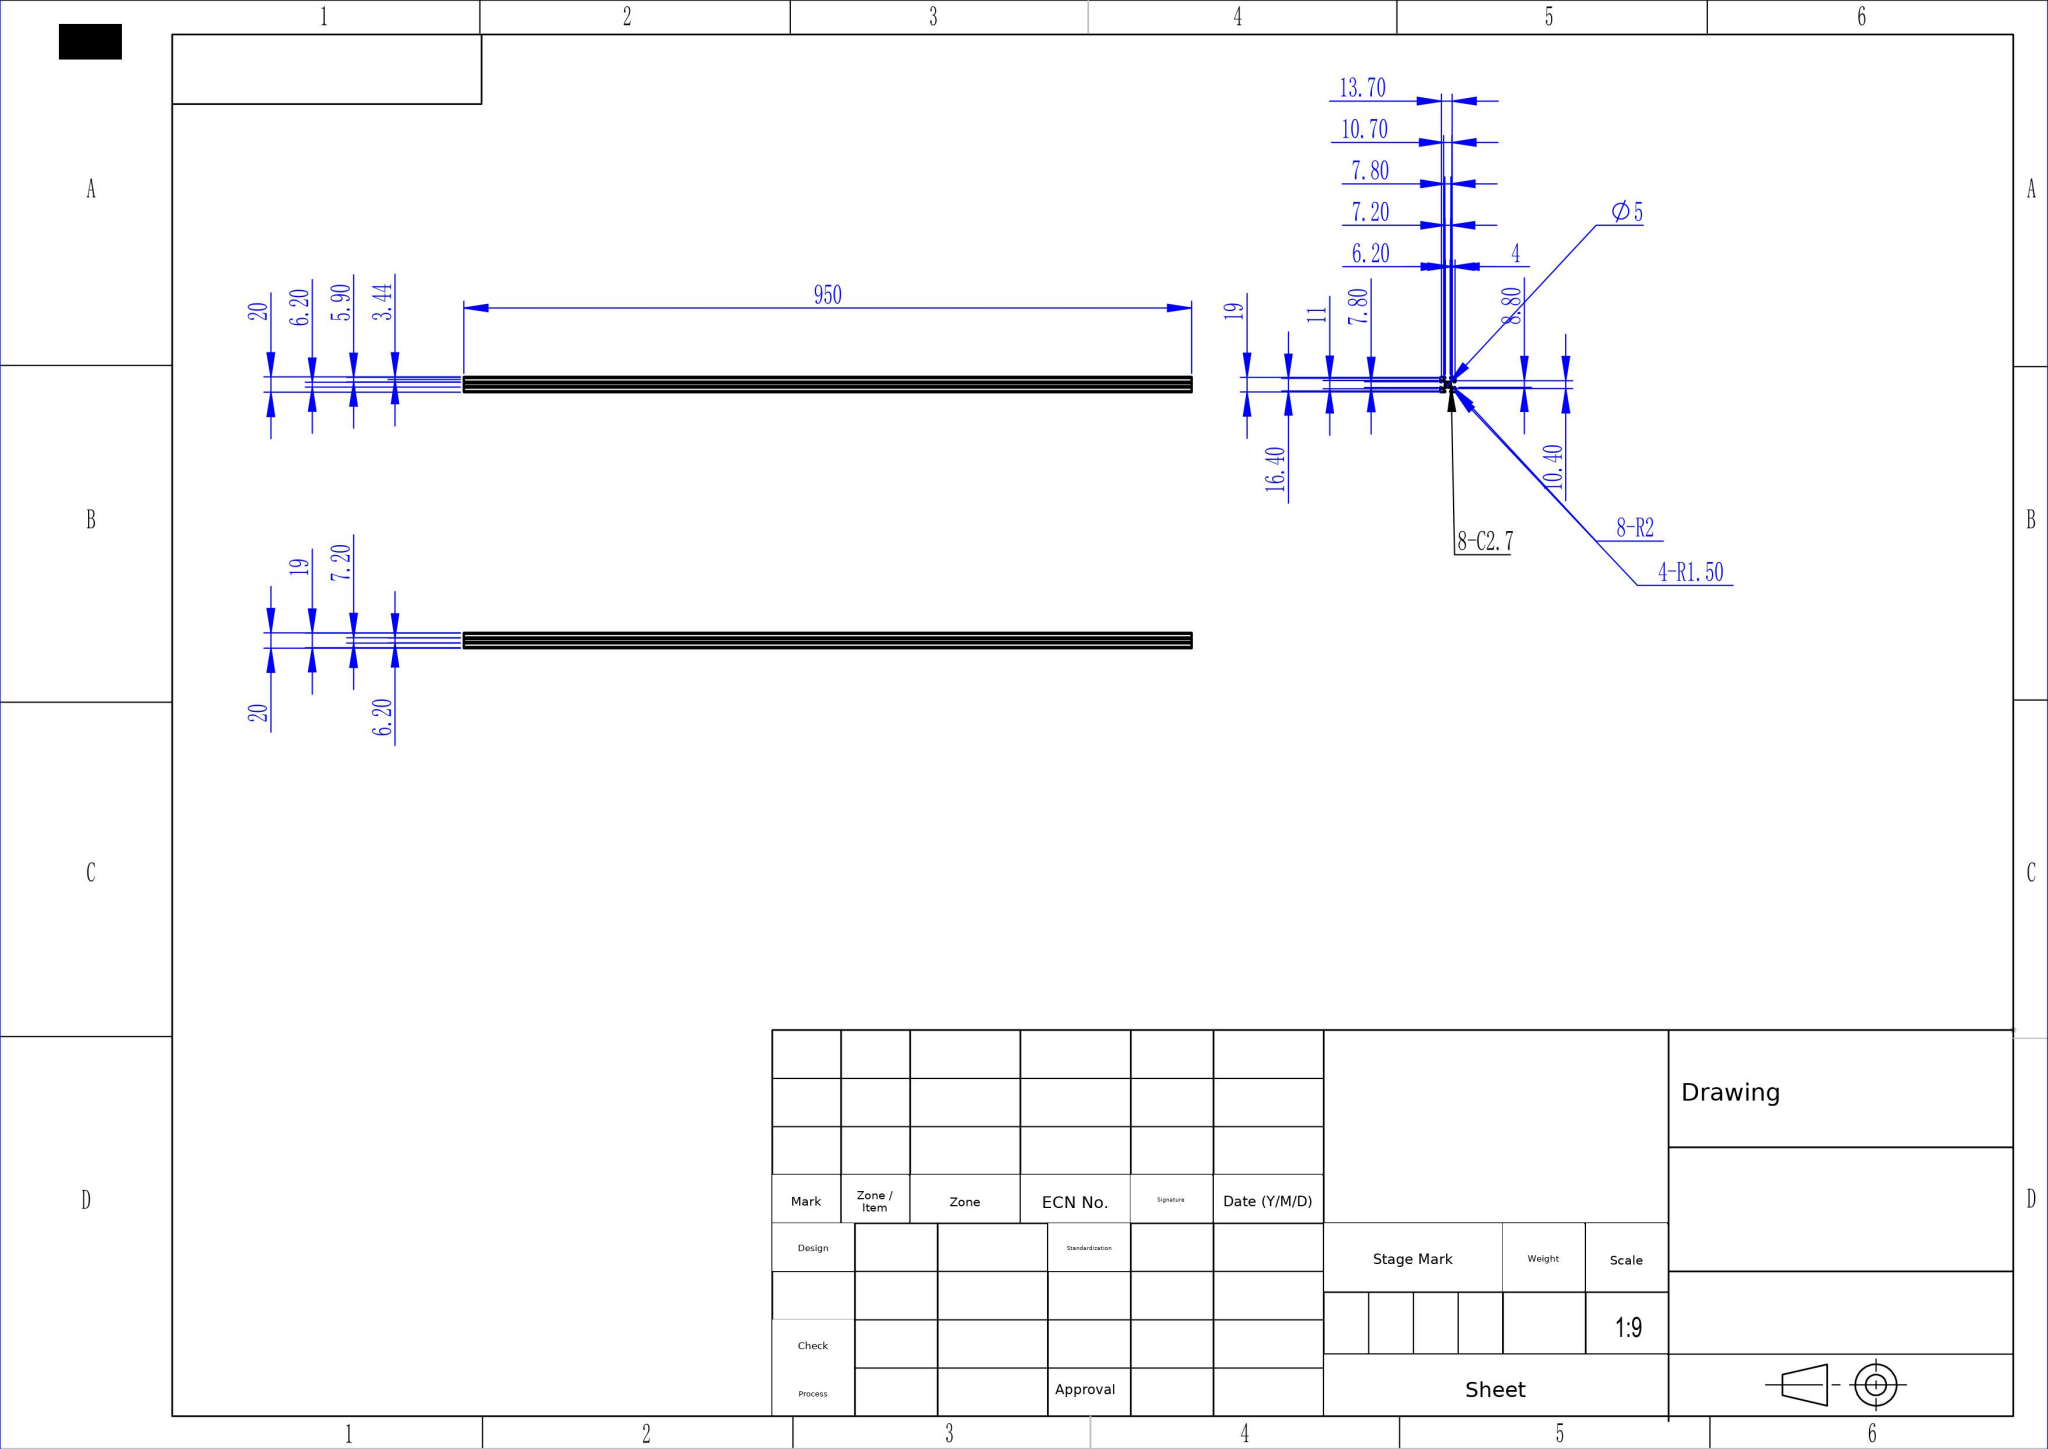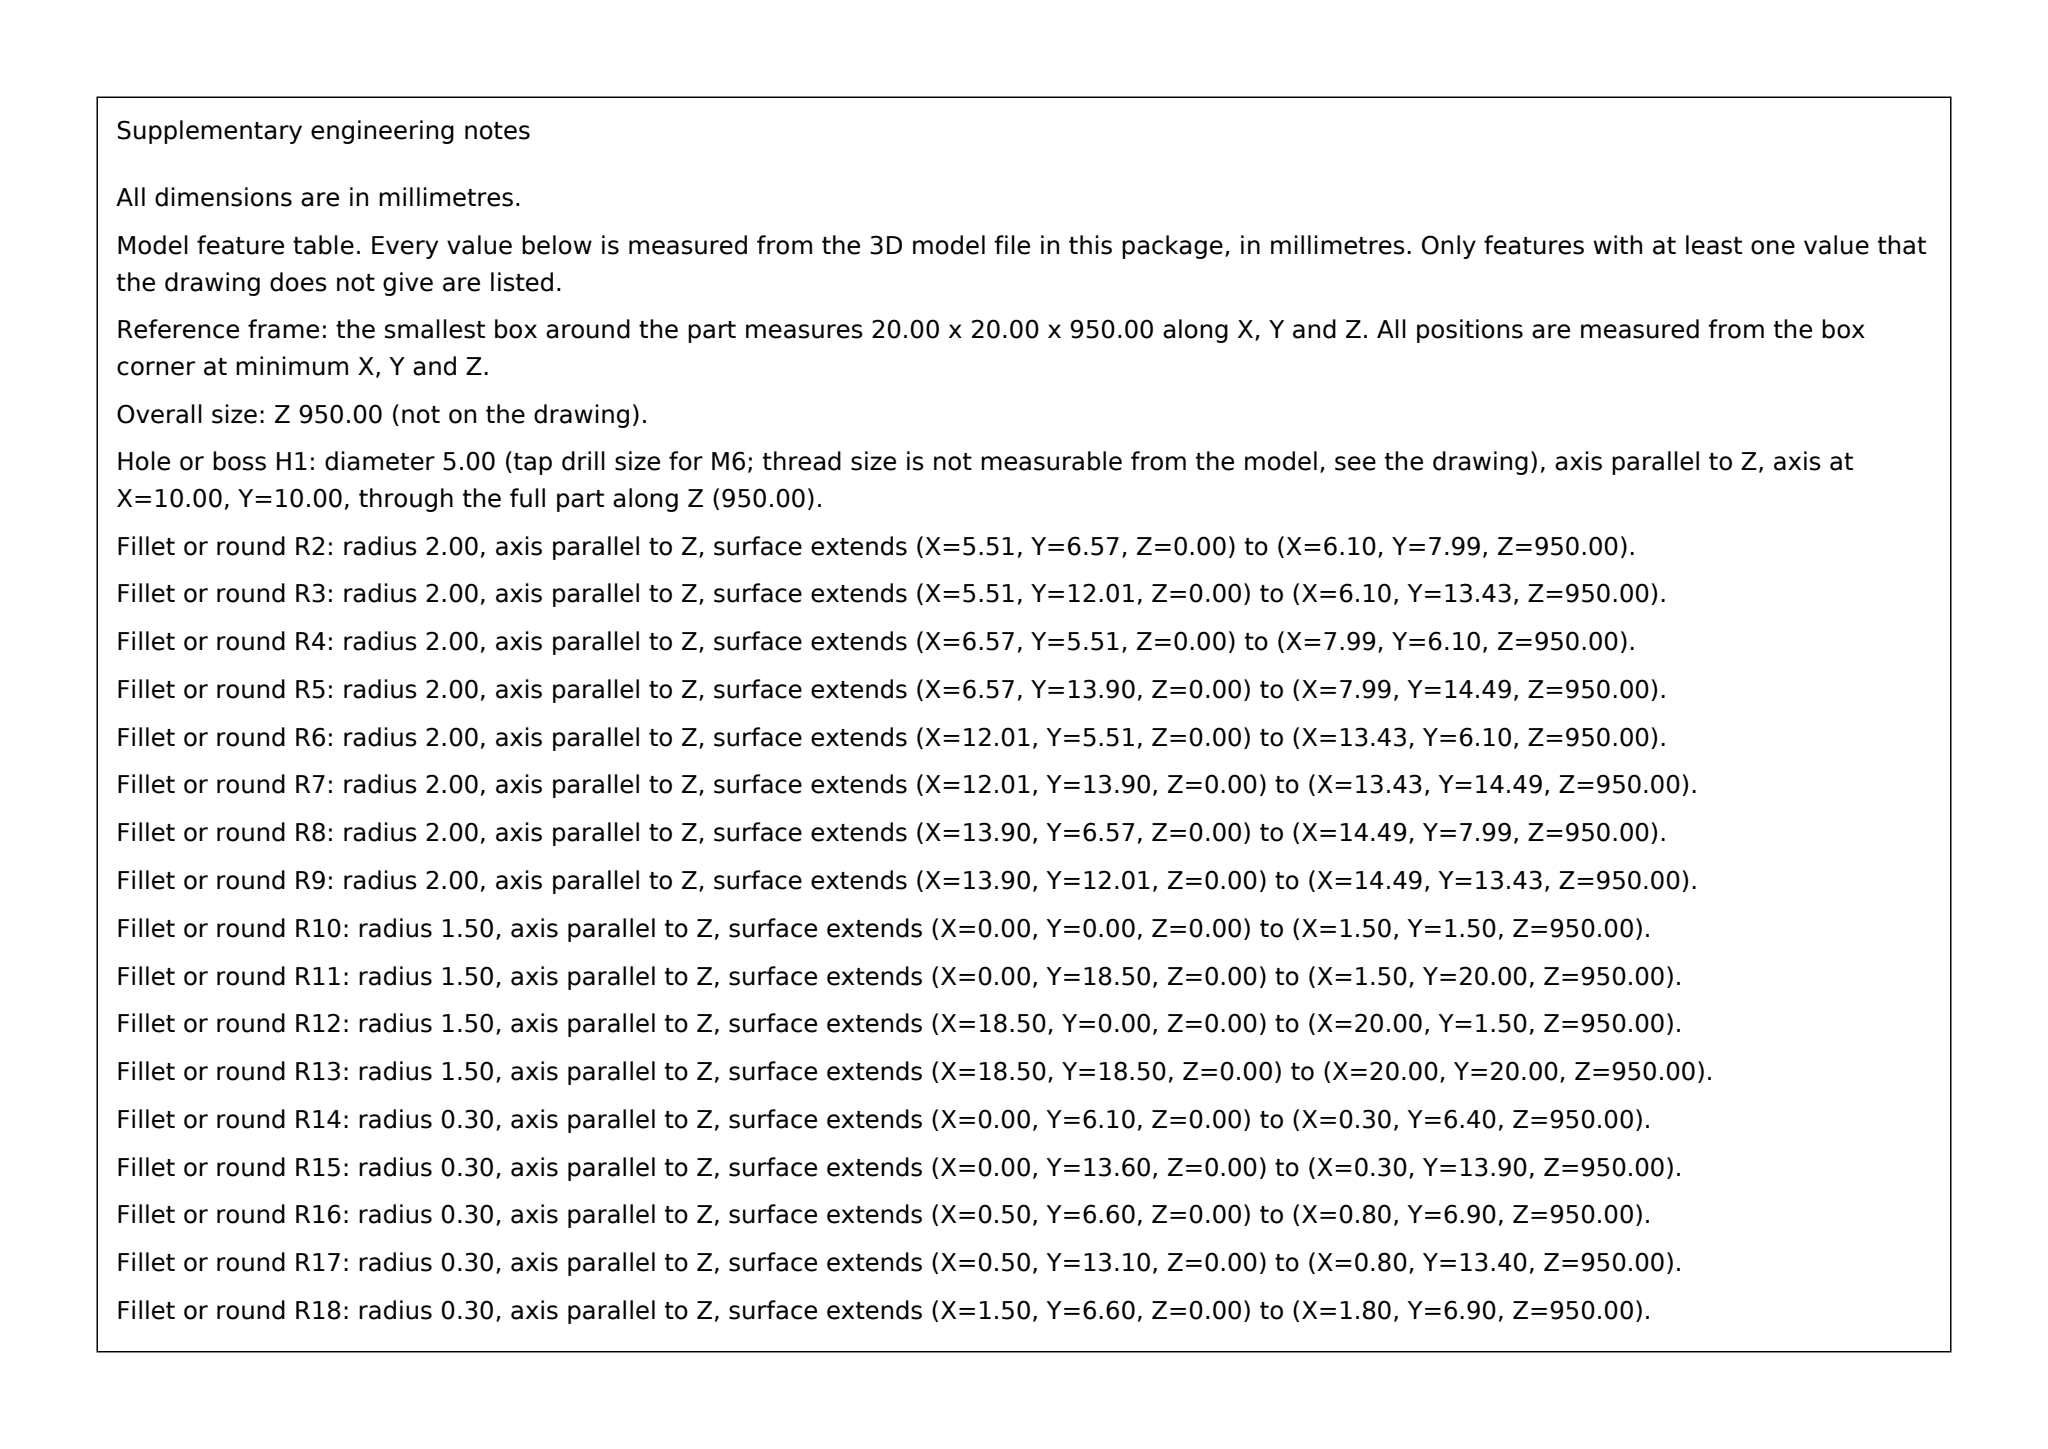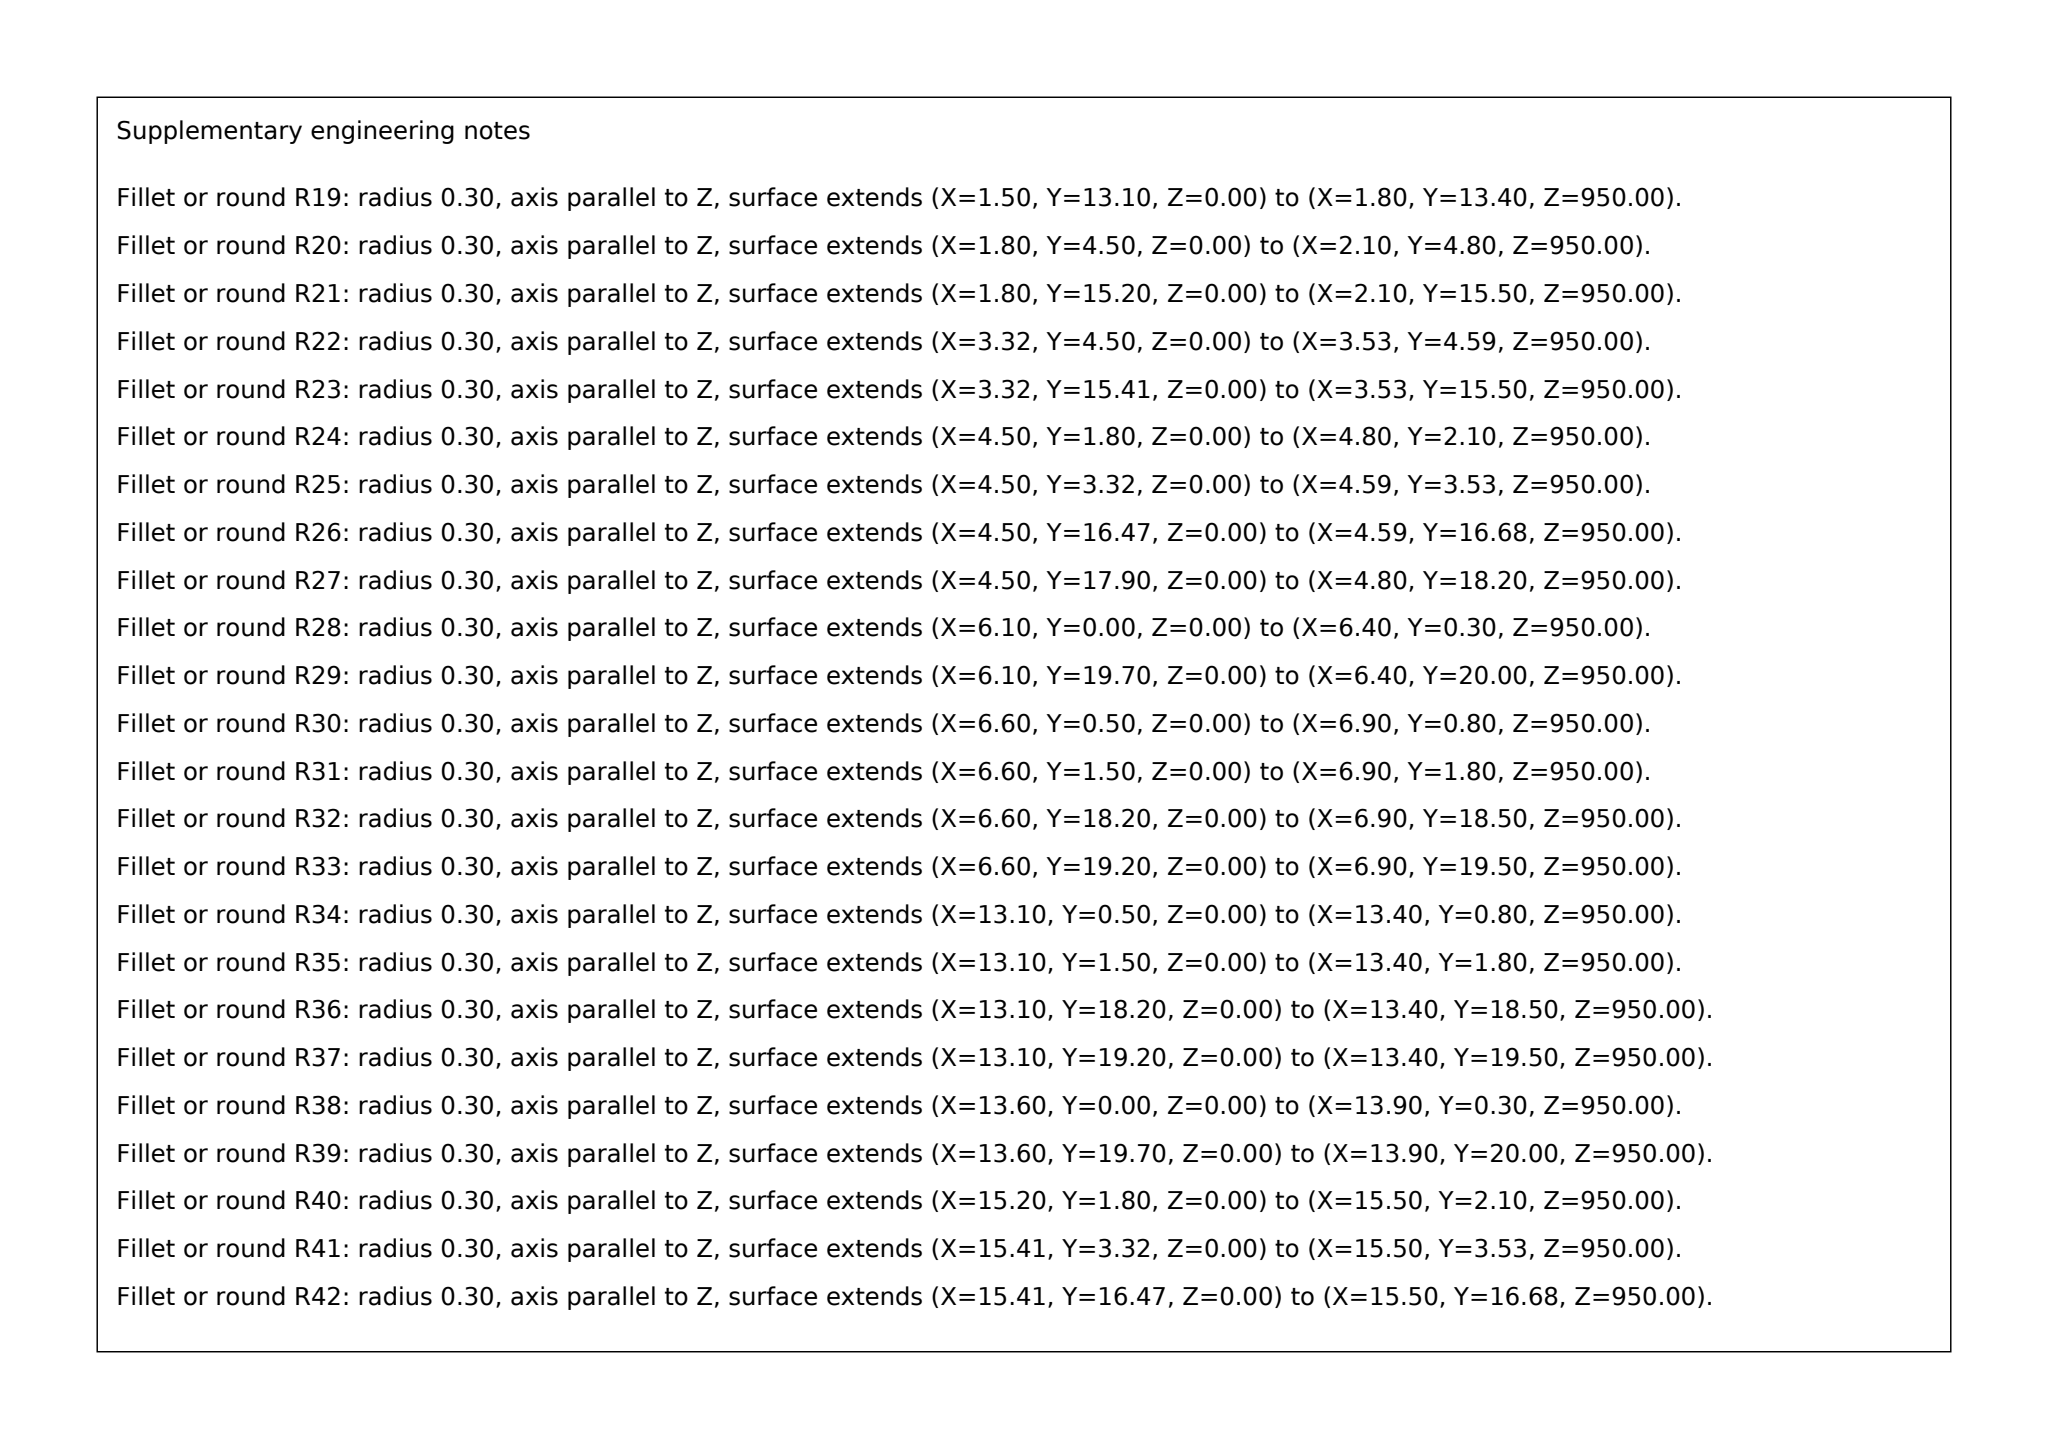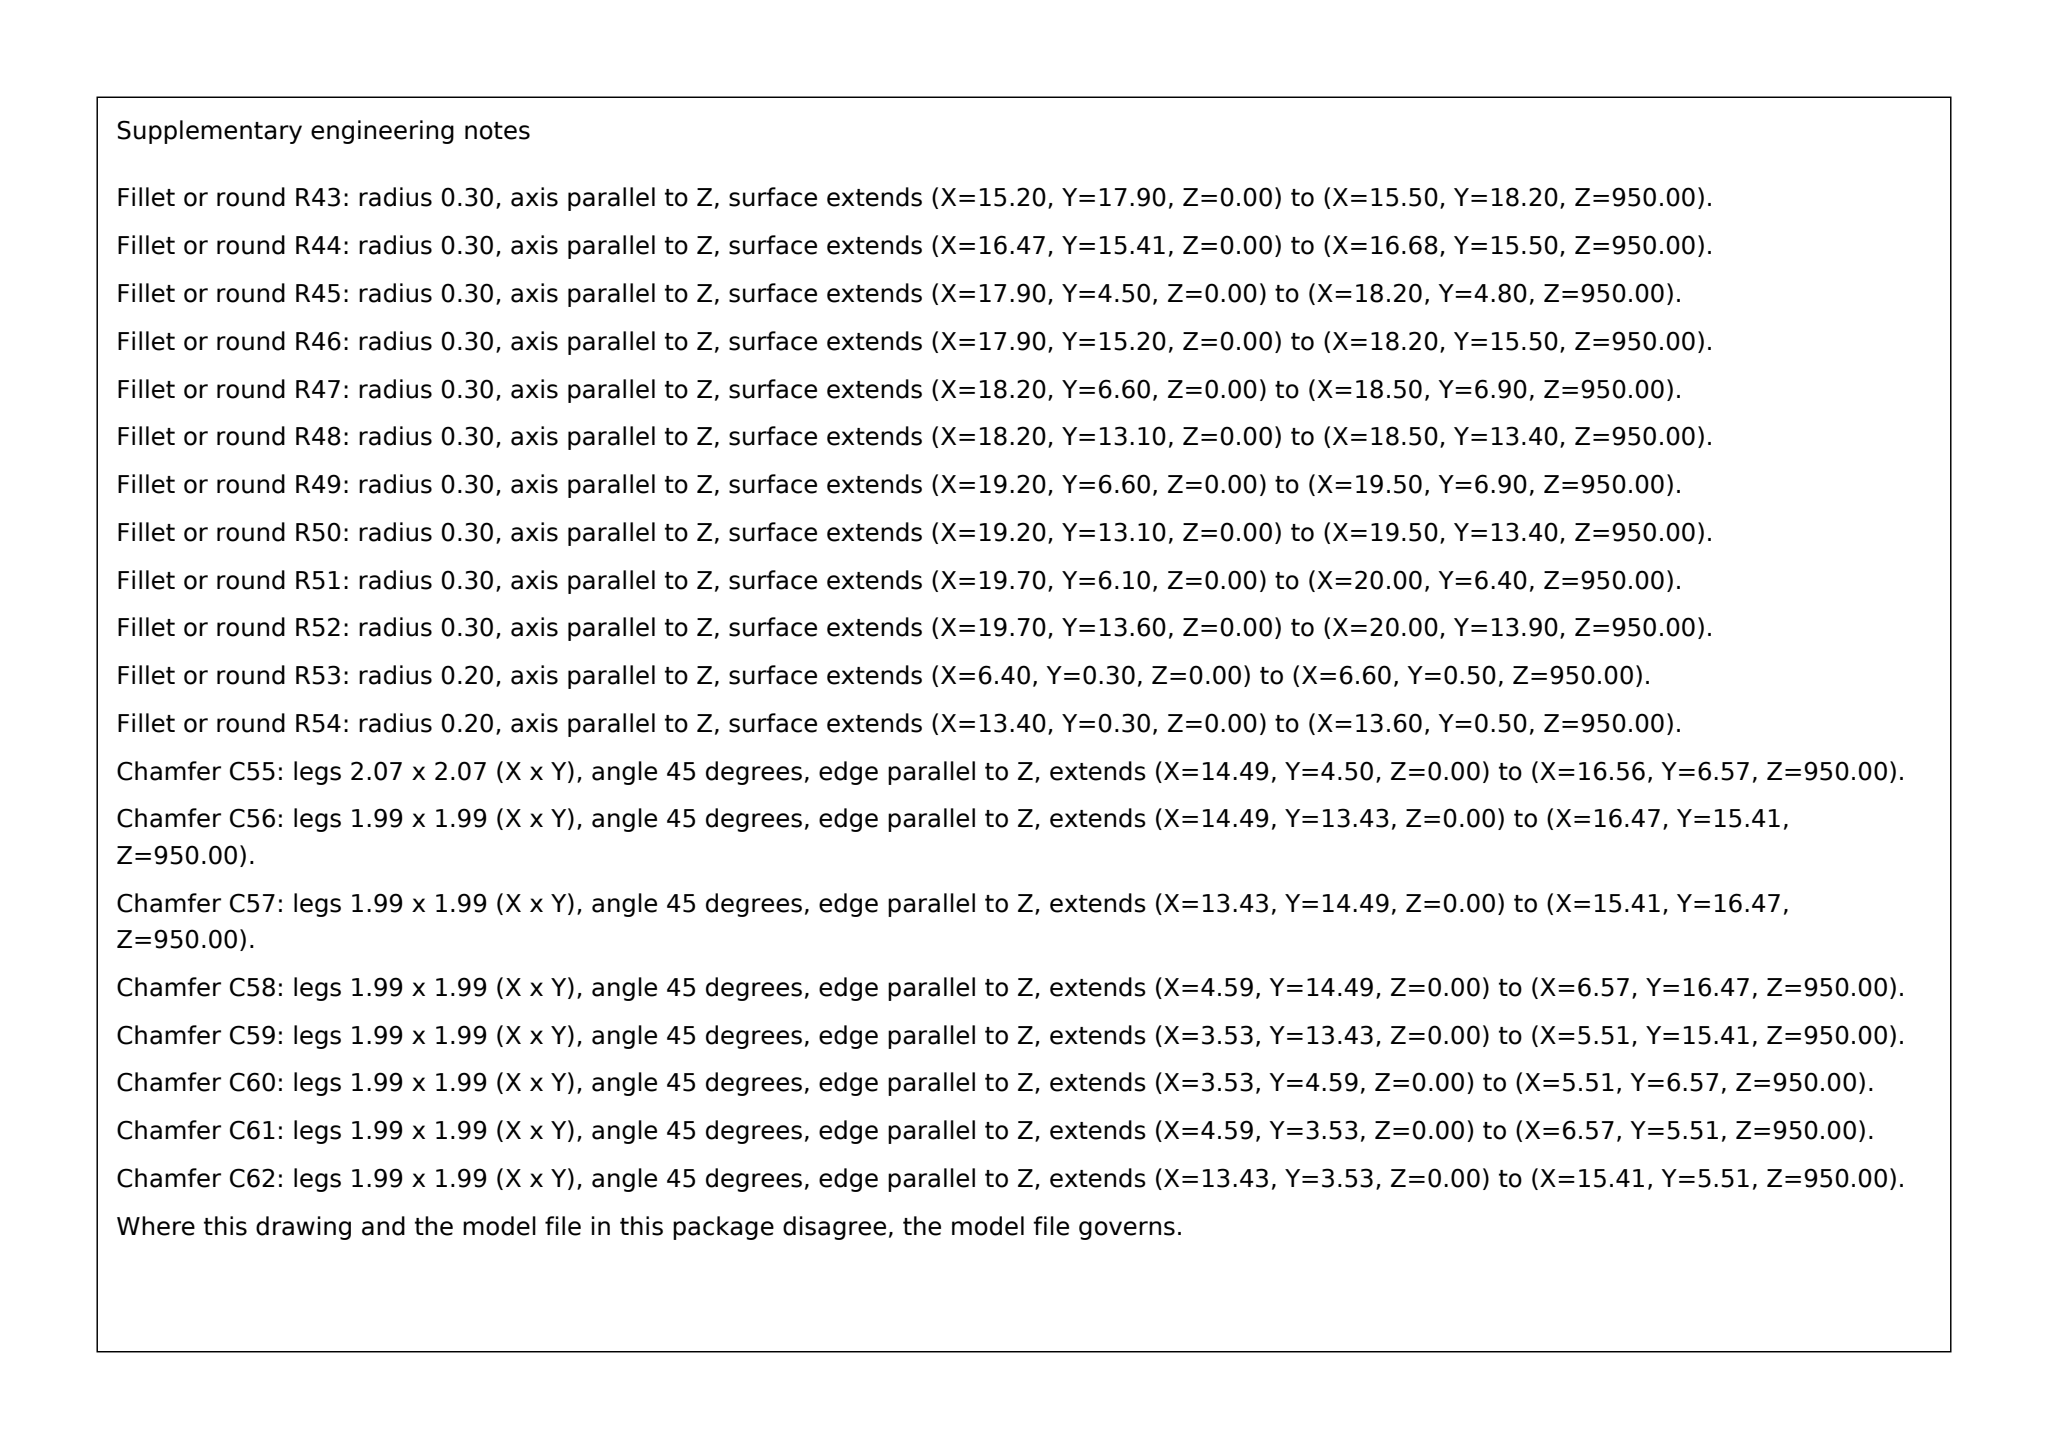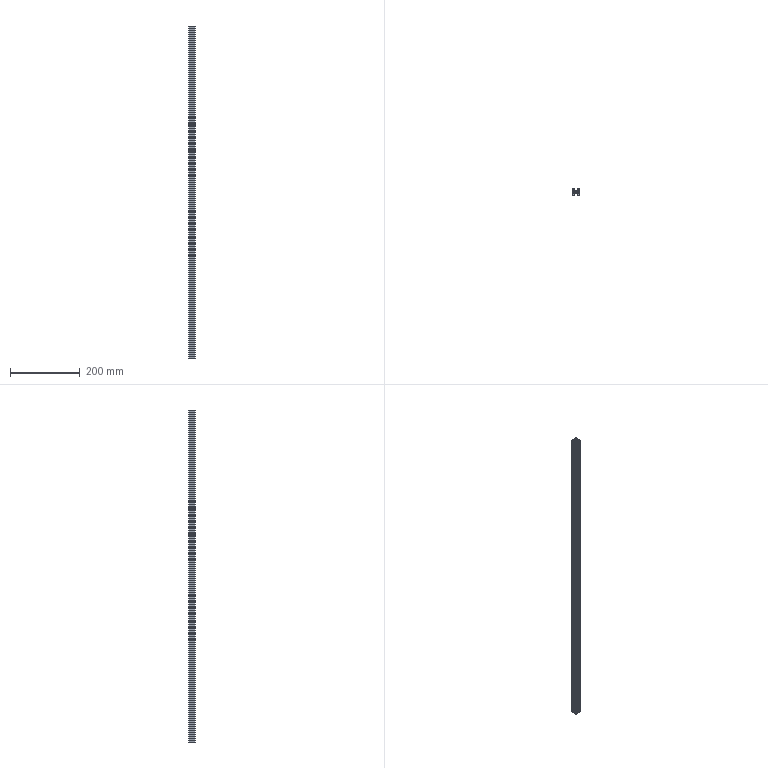Part | SolidWorks | mm | 1 solid | 113 faces | box 20 x 20 x 950 mm | volume 162754 mm3 | plane 58 | cylinder 55 | commonest cylinder face diameters 0.6 x39 4 x8 3 x4 5 x2 0.4 x2
build123d program:
from build123d import *

# Parameters (mm, degrees)
SKETCH1_R           = 2.5
BOSS_EXTRUDE1_DEPTH = 950


with BuildPart() as part:
    # Sketch1 → Boss-Extrude1 (new body)
    with BuildSketch(Plane(origin=(0, 0, 0), x_dir=(-1, 0, 0), z_dir=(0, 0, -1))):
        with BuildLine():
            Line((-5845.236, 2818.35), (-5845.236, 2820.15))
            ThreePointArc((-5845.236, 2820.15), (-5845.323, 2820.362), (-5845.536, 2820.45))
            Line((-5845.536, 2820.45), (-5846.236, 2820.45))
            ThreePointArc((-5846.236, 2820.45), (-5846.448, 2820.362), (-5846.536, 2820.15))
            Line((-5846.536, 2820.15), (-5846.536, 2819.95))
            Line((-5846.536, 2819.95), (-5846.736, 2819.95))
            ThreePointArc((-5846.736, 2819.95), (-5846.948, 2819.862), (-5847.036, 2819.65))
            Line((-5847.036, 2819.65), (-5847.036, 2815.05))
            ThreePointArc((-5847.036, 2815.05), (-5846.596, 2813.989), (-5845.536, 2813.55))
            Line((-5845.536, 2813.55), (-5840.936, 2813.55))
            ThreePointArc((-5840.936, 2813.55), (-5840.723, 2813.638), (-5840.636, 2813.85))
            ThreePointArc((-5840.636, 2813.85), (-5840.577, 2813.991), (-5840.436, 2814.05))
            ThreePointArc((-5840.436, 2814.05), (-5840.223, 2814.138), (-5840.136, 2814.35))
            Line((-5840.136, 2814.35), (-5840.136, 2815.05))
            ThreePointArc((-5840.136, 2815.05), (-5840.223, 2815.262), (-5840.436, 2815.35))
            Line((-5840.436, 2815.35), (-5842.236, 2815.35))
            ThreePointArc((-5842.236, 2815.35), (-5842.448, 2815.438), (-5842.536, 2815.65))
            Line((-5842.536, 2815.65), (-5842.536, 2816.865))
            ThreePointArc((-5842.536, 2816.865), (-5842.513, 2816.98), (-5842.448, 2817.077))
            Line((-5842.448, 2817.077), (-5840.461, 2819.064))
            ThreePointArc((-5840.461, 2819.064), (-5839.812, 2819.498), (-5839.046, 2819.65))
            Line((-5839.046, 2819.65), (-5835.025, 2819.65))
            ThreePointArc((-5835.025, 2819.65), (-5834.259, 2819.498), (-5833.61, 2819.064))
            Line((-5833.61, 2819.064), (-5831.623, 2817.077))
            ThreePointArc((-5831.623, 2817.077), (-5831.558, 2816.98), (-5831.536, 2816.865))
            Line((-5831.536, 2816.865), (-5831.536, 2815.65))
            ThreePointArc((-5831.536, 2815.65), (-5831.623, 2815.438), (-5831.836, 2815.35))
            Line((-5831.836, 2815.35), (-5833.636, 2815.35))
            ThreePointArc((-5833.636, 2815.35), (-5833.848, 2815.262), (-5833.936, 2815.05))
            Line((-5833.936, 2815.05), (-5833.936, 2814.35))
            ThreePointArc((-5833.936, 2814.35), (-5833.848, 2814.138), (-5833.636, 2814.05))
            ThreePointArc((-5833.636, 2814.05), (-5833.494, 2813.991), (-5833.436, 2813.85))
            ThreePointArc((-5833.436, 2813.85), (-5833.348, 2813.638), (-5833.136, 2813.55))
            Line((-5833.136, 2813.55), (-5828.536, 2813.55))
            ThreePointArc((-5828.536, 2813.55), (-5827.475, 2813.989), (-5827.036, 2815.05))
            Line((-5827.036, 2815.05), (-5827.036, 2819.65))
            ThreePointArc((-5827.036, 2819.65), (-5827.123, 2819.862), (-5827.336, 2819.95))
            Line((-5827.336, 2819.95), (-5827.536, 2819.95))
            Line((-5827.536, 2819.95), (-5827.536, 2820.15))
            ThreePointArc((-5827.536, 2820.15), (-5827.623, 2820.362), (-5827.836, 2820.45))
            Line((-5827.836, 2820.45), (-5828.536, 2820.45))
            ThreePointArc((-5828.536, 2820.45), (-5828.748, 2820.362), (-5828.836, 2820.15))
            Line((-5828.836, 2820.15), (-5828.836, 2818.35))
            ThreePointArc((-5828.836, 2818.35), (-5828.923, 2818.138), (-5829.136, 2818.05))
            Line((-5829.136, 2818.05), (-5830.351, 2818.05))
            ThreePointArc((-5830.351, 2818.05), (-5830.465, 2818.073), (-5830.563, 2818.138))
            Line((-5830.563, 2818.138), (-5832.55, 2820.125))
            ThreePointArc((-5832.55, 2820.125), (-5832.983, 2820.774), (-5833.136, 2821.539))
            Line((-5833.136, 2821.539), (-5833.136, 2825.561))
            ThreePointArc((-5833.136, 2825.561), (-5832.983, 2826.326), (-5832.55, 2826.975))
            Line((-5832.55, 2826.975), (-5830.563, 2828.962))
            ThreePointArc((-5830.563, 2828.962), (-5830.465, 2829.027), (-5830.351, 2829.05))
            Line((-5830.351, 2829.05), (-5829.136, 2829.05))
            ThreePointArc((-5829.136, 2829.05), (-5828.923, 2828.962), (-5828.836, 2828.75))
            Line((-5828.836, 2828.75), (-5828.836, 2826.95))
            ThreePointArc((-5828.836, 2826.95), (-5828.748, 2826.738), (-5828.536, 2826.65))
            Line((-5828.536, 2826.65), (-5827.836, 2826.65))
            ThreePointArc((-5827.836, 2826.65), (-5827.623, 2826.738), (-5827.536, 2826.95))
            Line((-5827.536, 2826.95), (-5827.536, 2827.15))
            Line((-5827.536, 2827.15), (-5827.336, 2827.15))
            ThreePointArc((-5827.336, 2827.15), (-5827.123, 2827.238), (-5827.036, 2827.45))
            Line((-5827.036, 2827.45), (-5827.036, 2832.05))
            ThreePointArc((-5827.036, 2832.05), (-5827.475, 2833.11), (-5828.536, 2833.55))
            Line((-5828.536, 2833.55), (-5833.136, 2833.55))
            ThreePointArc((-5833.136, 2833.55), (-5833.348, 2833.462), (-5833.436, 2833.25))
            Line((-5833.436, 2833.25), (-5833.436, 2833.05))
            Line((-5833.436, 2833.05), (-5833.636, 2833.05))
            ThreePointArc((-5833.636, 2833.05), (-5833.848, 2832.962), (-5833.936, 2832.75))
            Line((-5833.936, 2832.75), (-5833.936, 2832.05))
            ThreePointArc((-5833.936, 2832.05), (-5833.848, 2831.838), (-5833.636, 2831.75))
            Line((-5833.636, 2831.75), (-5831.836, 2831.75))
            ThreePointArc((-5831.836, 2831.75), (-5831.623, 2831.662), (-5831.536, 2831.45))
            Line((-5831.536, 2831.45), (-5831.536, 2830.235))
            ThreePointArc((-5831.536, 2830.235), (-5831.558, 2830.12), (-5831.623, 2830.023))
            Line((-5831.623, 2830.023), (-5833.61, 2828.036))
            ThreePointArc((-5833.61, 2828.036), (-5834.259, 2827.602), (-5835.025, 2827.45))
            Line((-5835.025, 2827.45), (-5839.046, 2827.45))
            ThreePointArc((-5839.046, 2827.45), (-5839.812, 2827.602), (-5840.461, 2828.036))
            Line((-5840.461, 2828.036), (-5842.448, 2830.023))
            ThreePointArc((-5842.448, 2830.023), (-5842.513, 2830.12), (-5842.536, 2830.235))
            Line((-5842.536, 2830.235), (-5842.536, 2831.45))
            ThreePointArc((-5842.536, 2831.45), (-5842.448, 2831.662), (-5842.236, 2831.75))
            Line((-5842.236, 2831.75), (-5840.436, 2831.75))
            ThreePointArc((-5840.436, 2831.75), (-5840.223, 2831.838), (-5840.136, 2832.05))
            Line((-5840.136, 2832.05), (-5840.136, 2832.75))
            ThreePointArc((-5840.136, 2832.75), (-5840.223, 2832.962), (-5840.436, 2833.05))
            Line((-5840.436, 2833.05), (-5840.636, 2833.05))
            Line((-5840.636, 2833.05), (-5840.636, 2833.25))
            ThreePointArc((-5840.636, 2833.25), (-5840.723, 2833.462), (-5840.936, 2833.55))
            Line((-5840.936, 2833.55), (-5845.536, 2833.55))
            ThreePointArc((-5845.536, 2833.55), (-5846.596, 2833.11), (-5847.036, 2832.05))
            Line((-5847.036, 2832.05), (-5847.036, 2827.45))
            ThreePointArc((-5847.036, 2827.45), (-5846.948, 2827.238), (-5846.736, 2827.15))
            Line((-5846.736, 2827.15), (-5846.536, 2827.15))
            Line((-5846.536, 2827.15), (-5846.536, 2826.95))
            ThreePointArc((-5846.536, 2826.95), (-5846.448, 2826.738), (-5846.236, 2826.65))
            Line((-5846.236, 2826.65), (-5845.536, 2826.65))
            ThreePointArc((-5845.536, 2826.65), (-5845.323, 2826.738), (-5845.236, 2826.95))
            Line((-5845.236, 2826.95), (-5845.236, 2828.75))
            ThreePointArc((-5845.236, 2828.75), (-5845.148, 2828.962), (-5844.936, 2829.05))
            Line((-5844.936, 2829.05), (-5843.72, 2829.05))
            ThreePointArc((-5843.72, 2829.05), (-5843.606, 2829.027), (-5843.508, 2828.962))
            Line((-5843.508, 2828.962), (-5841.521, 2826.975))
            ThreePointArc((-5841.521, 2826.975), (-5841.088, 2826.326), (-5840.936, 2825.561))
            Line((-5840.936, 2825.561), (-5840.936, 2821.539))
            ThreePointArc((-5840.936, 2821.539), (-5841.088, 2820.774), (-5841.521, 2820.125))
            Line((-5841.521, 2820.125), (-5843.596, 2818.05))
            Line((-5843.596, 2818.05), (-5844.936, 2818.05))
            ThreePointArc((-5844.936, 2818.05), (-5845.148, 2818.138), (-5845.236, 2818.35))
        make_face()
        with Locations((-5837.036, 2823.55)):
            Circle(SKETCH1_R, mode=Mode.SUBTRACT)
    extrude(amount=-BOSS_EXTRUDE1_DEPTH)


solid = part.part